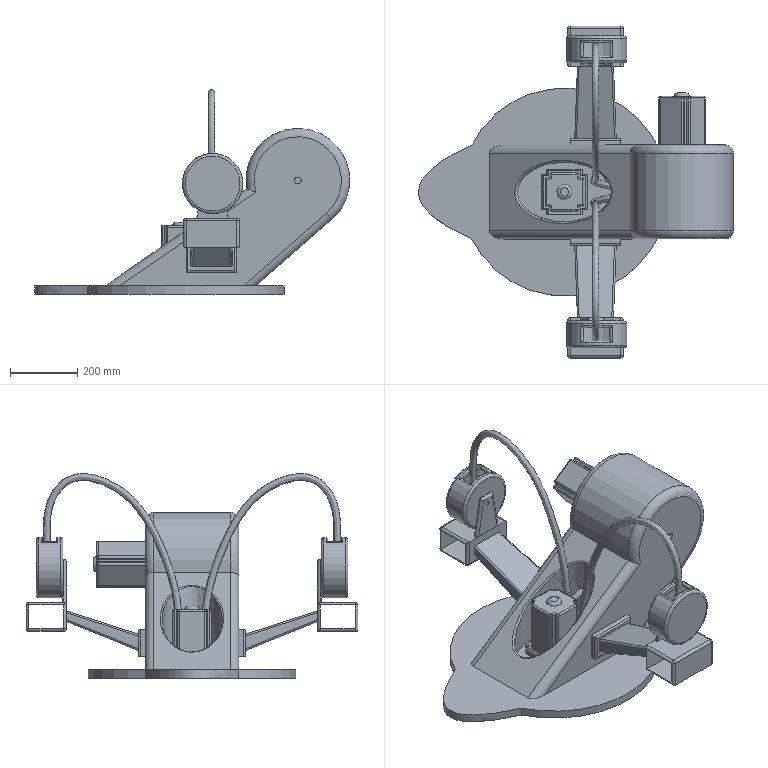Component | NX | 2_SHOULDER_ROTATOR | 16 solids | 345 faces | volume 56115785 mm3 | plane 171 | cylinder 116 | sphere 23 | torus 20 | cone 8 | spline 5 | other 2 | commonest cylinder face diameters 10 x70 16 x25 29.8 x8 50 x4 180 x3 20 x2 310 x1 160 x1